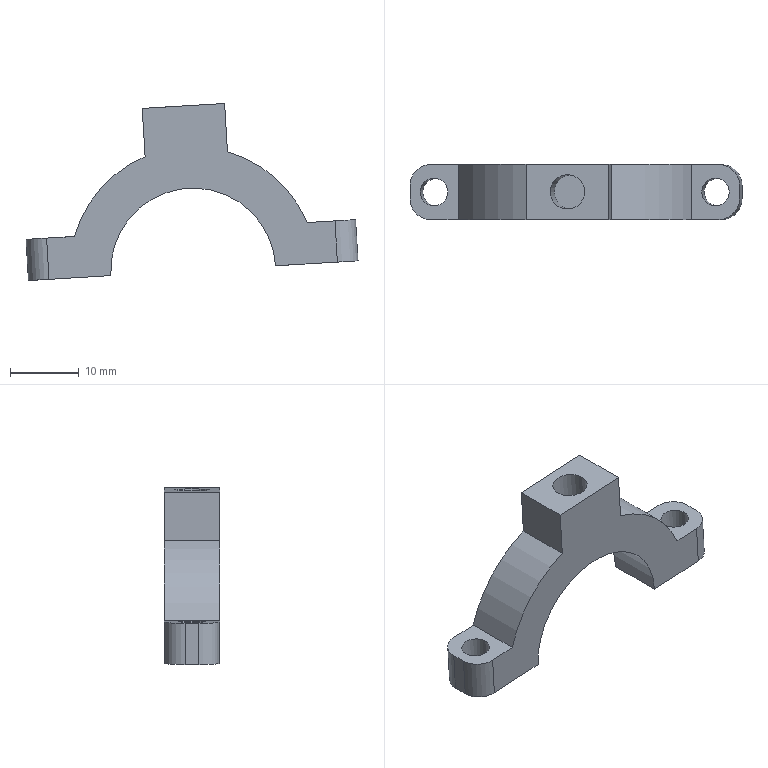Component | NX | UPPER_PISTON_RING | 1 solid | 22 faces | volume 3086 mm3 | plane 12 | cylinder 10 | commonest cylinder face diameters 6 x4 36 x2 4 x2 24 x1 5 x1